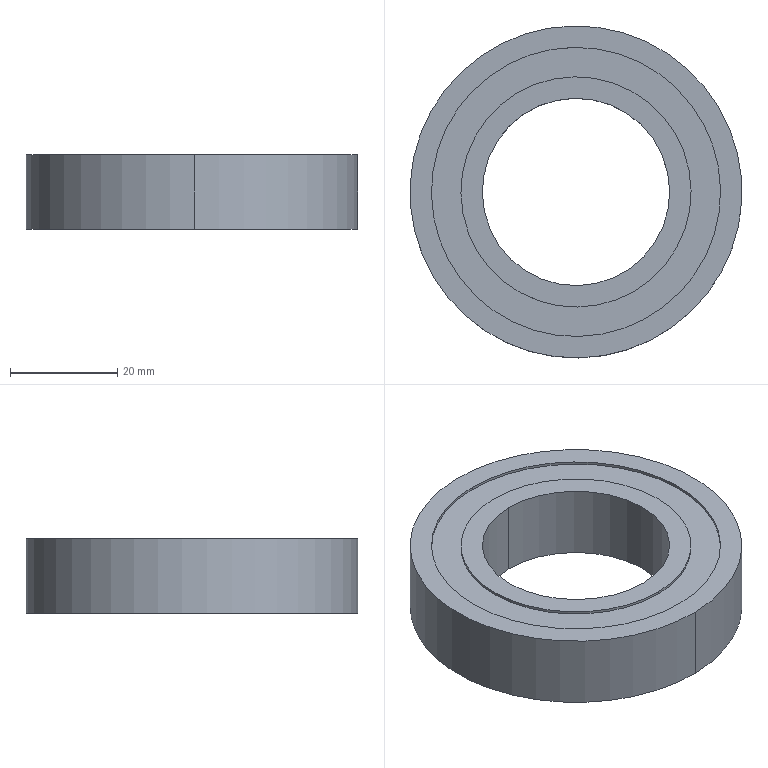Component | SolidWorks | DeepGrooveBallBearing6007-1 | 1 solid | 18 faces | box 62 x 62 x 14 mm | volume 27959 mm3 | cylinder 12 | plane 6 | commonest cylinder face diameters 54 x4 43 x4 62 x2 35 x2 | material A3
build123d program:
from build123d import *


with BuildPart() as part:
    # Sketch1 → Revolve1 (revolve)
    with BuildSketch(Plane(origin=(0, 0, 0), x_dir=(1, 0, 0), z_dir=(0, 1, 0)), mode=Mode.PRIVATE) as revolve1_sk:
        Polygon((-31, -7), (-31, 7), (-27, 7), (-27, 6.5), (-21.5, 6.5), (-21.5, 7), (-17.5, 7), (-17.5, -7), (-21.5, -7), (-21.5, -6.5), (-27, -6.5), (-27, -7), align=None)
    revolve(revolve1_sk.sketch.rotate(Axis((0, 0, 0), (0, 0, -1)), 180), axis=Axis((0, 0, 0), (0, 0, -1)))


solid = part.part

# Placed as in the assembly
solid = solid.moved(Location((733.029, 200.722, 14.5), (0, 0, 0)))
STEP:
#1=COLOUR_RGB('',0.7922,0.8196,0.9333);
#2=FILL_AREA_STYLE_COLOUR('',#1);
#3=FILL_AREA_STYLE('',(#2));
#4=SURFACE_STYLE_FILL_AREA(#3);
#5=SURFACE_SIDE_STYLE('',(#4));
#6=SURFACE_STYLE_USAGE(.BOTH.,#5);
#7=PRESENTATION_STYLE_ASSIGNMENT((#6));
#8=CARTESIAN_POINT('',(28.879,6.682,0.8465));
#9=VERTEX_POINT('',#8);
#10=CARTESIAN_POINT('',(28.839,9.123,0.8465));
#11=VERTEX_POINT('',#10);
#12=CARTESIAN_POINT('',(28.859,7.902,0.8465));
#13=DIRECTION('',(-0.,-0.,-1.));
#14=DIRECTION('',(0.01645,-0.9999,0.));
#15=AXIS2_PLACEMENT_3D('',#12,#13,#14);
#16=CIRCLE('',#15,1.22);
#17=EDGE_CURVE('',#9,#11,#16,.T.);
#18=ORIENTED_EDGE('',*,*,#17,.T.);
#19=CARTESIAN_POINT('',(28.839,9.123,0.2953));
#20=VERTEX_POINT('',#19);
#21=CARTESIAN_POINT('',(28.839,9.123,0.5709));
#22=DIRECTION('',(-0.,-0.,-1.));
#23=VECTOR('',#22,39.37);
#24=LINE('',#21,#23);
#25=EDGE_CURVE('',#11,#20,#24,.T.);
#26=ORIENTED_EDGE('',*,*,#25,.T.);
#27=CARTESIAN_POINT('',(28.879,6.682,0.2953));
#28=VERTEX_POINT('',#27);
#29=CARTESIAN_POINT('',(28.859,7.902,0.2953));
#30=DIRECTION('',(-0.,-0.,-1.));
#31=DIRECTION('',(0.01645,-0.9999,0.));
#32=AXIS2_PLACEMENT_3D('',#29,#30,#31);
#33=CIRCLE('',#32,1.22);
#34=EDGE_CURVE('',#28,#20,#33,.T.);
#35=ORIENTED_EDGE('',*,*,#34,.F.);
#36=CARTESIAN_POINT('',(28.879,6.682,0.5709));
#37=DIRECTION('',(-0.,-0.,-1.));
#38=VECTOR('',#37,39.37);
#39=LINE('',#36,#38);
#40=EDGE_CURVE('',#9,#28,#39,.T.);
#41=ORIENTED_EDGE('',*,*,#40,.F.);
#42=EDGE_LOOP('',(#18,#26,#35,#41));
#43=FACE_OUTER_BOUND('',#42,.T.);
#44=CARTESIAN_POINT('',(28.859,7.902,0.5709));
#45=DIRECTION('',(-0.,-0.,-1.));
#46=DIRECTION('',(0.01645,-0.9999,0.));
#47=AXIS2_PLACEMENT_3D('',#44,#45,#46);
#48=CYLINDRICAL_SURFACE('',#47,1.22);
#49=ADVANCED_FACE('',(#43),#48,.T.);
#50=CARTESIAN_POINT('',(28.842,8.965,0.315));
#51=VERTEX_POINT('',#50);
#52=CARTESIAN_POINT('',(28.877,6.84,0.315));
#53=VERTEX_POINT('',#52);
#54=CARTESIAN_POINT('',(28.859,7.902,0.315));
#55=DIRECTION('',(-0.,-0.,-1.));
#56=DIRECTION('',(0.01645,-0.9999,0.));
#57=AXIS2_PLACEMENT_3D('',#54,#55,#56);
#58=CIRCLE('',#57,1.063);
#59=EDGE_CURVE('',#51,#53,#58,.T.);
#60=ORIENTED_EDGE('',*,*,#59,.F.);
#61=CARTESIAN_POINT('',(28.842,8.965,0.2953));
#62=VERTEX_POINT('',#61);
#63=CARTESIAN_POINT('',(28.842,8.965,0.5709));
#64=DIRECTION('',(-0.,-0.,-1.));
#65=VECTOR('',#64,39.37);
#66=LINE('',#63,#65);
#67=EDGE_CURVE('',#51,#62,#66,.T.);
#68=ORIENTED_EDGE('',*,*,#67,.T.);
#69=CARTESIAN_POINT('',(28.877,6.84,0.2953));
#70=VERTEX_POINT('',#69);
#71=CARTESIAN_POINT('',(28.859,7.902,0.2953));
#72=DIRECTION('',(-0.,-0.,-1.));
#73=DIRECTION('',(0.01645,-0.9999,0.));
#74=AXIS2_PLACEMENT_3D('',#71,#72,#73);
#75=CIRCLE('',#74,1.063);
#76=EDGE_CURVE('',#62,#70,#75,.T.);
#77=ORIENTED_EDGE('',*,*,#76,.T.);
#78=CARTESIAN_POINT('',(28.877,6.84,0.5709));
#79=DIRECTION('',(-0.,-0.,-1.));
#80=VECTOR('',#79,39.37);
#81=LINE('',#78,#80);
#82=EDGE_CURVE('',#53,#70,#81,.T.);
#83=ORIENTED_EDGE('',*,*,#82,.F.);
#84=EDGE_LOOP('',(#60,#68,#77,#83));
#85=FACE_OUTER_BOUND('',#84,.T.);
#86=CARTESIAN_POINT('',(28.859,7.902,0.5709));
#87=DIRECTION('',(-0.,-0.,-1.));
#88=DIRECTION('',(0.01645,-0.9999,0.));
#89=AXIS2_PLACEMENT_3D('',#86,#87,#88);
#90=CYLINDRICAL_SURFACE('',#89,1.063);
#91=ADVANCED_FACE('',(#85),#90,.F.);
#92=CARTESIAN_POINT('',(28.873,7.056,0.315));
#93=VERTEX_POINT('',#92);
#94=CARTESIAN_POINT('',(28.845,8.749,0.315));
#95=VERTEX_POINT('',#94);
#96=CARTESIAN_POINT('',(28.859,7.902,0.315));
#97=DIRECTION('',(-0.,-0.,-1.));
#98=DIRECTION('',(0.01645,-0.9999,0.));
#99=AXIS2_PLACEMENT_3D('',#96,#97,#98);
#100=CIRCLE('',#99,0.8465);
#101=EDGE_CURVE('',#93,#95,#100,.T.);
#102=ORIENTED_EDGE('',*,*,#101,.T.);
#103=CARTESIAN_POINT('',(28.845,8.749,0.2953));
#104=VERTEX_POINT('',#103);
#105=CARTESIAN_POINT('',(28.845,8.749,0.5709));
#106=DIRECTION('',(-0.,-0.,-1.));
#107=VECTOR('',#106,39.37);
#108=LINE('',#105,#107);
#109=EDGE_CURVE('',#95,#104,#108,.T.);
#110=ORIENTED_EDGE('',*,*,#109,.T.);
#111=CARTESIAN_POINT('',(28.873,7.056,0.2953));
#112=VERTEX_POINT('',#111);
#113=CARTESIAN_POINT('',(28.859,7.902,0.2953));
#114=DIRECTION('',(-0.,-0.,-1.));
#115=DIRECTION('',(0.01645,-0.9999,0.));
#116=AXIS2_PLACEMENT_3D('',#113,#114,#115);
#117=CIRCLE('',#116,0.8465);
#118=EDGE_CURVE('',#112,#104,#117,.T.);
#119=ORIENTED_EDGE('',*,*,#118,.F.);
#120=CARTESIAN_POINT('',(28.873,7.056,0.5709));
#121=DIRECTION('',(-0.,-0.,-1.));
#122=VECTOR('',#121,39.37);
#123=LINE('',#120,#122);
#124=EDGE_CURVE('',#93,#112,#123,.T.);
#125=ORIENTED_EDGE('',*,*,#124,.F.);
#126=EDGE_LOOP('',(#102,#110,#119,#125));
#127=FACE_OUTER_BOUND('',#126,.T.);
#128=CARTESIAN_POINT('',(28.859,7.902,0.5709));
#129=DIRECTION('',(-0.,-0.,-1.));
#130=DIRECTION('',(0.01645,-0.9999,0.));
#131=AXIS2_PLACEMENT_3D('',#128,#129,#130);
#132=CYLINDRICAL_SURFACE('',#131,0.8465);
#133=ADVANCED_FACE('',(#127),#132,.T.);
#134=CARTESIAN_POINT('',(28.848,8.591,0.8465));
#135=VERTEX_POINT('',#134);
#136=CARTESIAN_POINT('',(28.871,7.214,0.8465));
#137=VERTEX_POINT('',#136);
#138=CARTESIAN_POINT('',(28.859,7.902,0.8465));
#139=DIRECTION('',(-0.,-0.,-1.));
#140=DIRECTION('',(0.01645,-0.9999,0.));
#141=AXIS2_PLACEMENT_3D('',#138,#139,#140);
#142=CIRCLE('',#141,0.689);
#143=EDGE_CURVE('',#135,#137,#142,.T.);
#144=ORIENTED_EDGE('',*,*,#143,.F.);
#145=CARTESIAN_POINT('',(28.848,8.591,0.2953));
#146=VERTEX_POINT('',#145);
#147=CARTESIAN_POINT('',(28.848,8.591,0.5709));
#148=DIRECTION('',(-0.,-0.,-1.));
#149=VECTOR('',#148,39.37);
#150=LINE('',#147,#149);
#151=EDGE_CURVE('',#135,#146,#150,.T.);
#152=ORIENTED_EDGE('',*,*,#151,.T.);
#153=CARTESIAN_POINT('',(28.871,7.214,0.2953));
#154=VERTEX_POINT('',#153);
#155=CARTESIAN_POINT('',(28.859,7.902,0.2953));
#156=DIRECTION('',(-0.,-0.,-1.));
#157=DIRECTION('',(0.01645,-0.9999,0.));
#158=AXIS2_PLACEMENT_3D('',#155,#156,#157);
#159=CIRCLE('',#158,0.689);
#160=EDGE_CURVE('',#146,#154,#159,.T.);
#161=ORIENTED_EDGE('',*,*,#160,.T.);
#162=CARTESIAN_POINT('',(28.871,7.214,0.5709));
#163=DIRECTION('',(-0.,-0.,-1.));
#164=VECTOR('',#163,39.37);
#165=LINE('',#162,#164);
#166=EDGE_CURVE('',#137,#154,#165,.T.);
#167=ORIENTED_EDGE('',*,*,#166,.F.);
#168=EDGE_LOOP('',(#144,#152,#161,#167));
#169=FACE_OUTER_BOUND('',#168,.T.);
#170=CARTESIAN_POINT('',(28.859,7.902,0.5709));
#171=DIRECTION('',(-0.,-0.,-1.));
#172=DIRECTION('',(0.01645,-0.9999,0.));
#173=AXIS2_PLACEMENT_3D('',#170,#171,#172);
#174=CYLINDRICAL_SURFACE('',#173,0.689);
#175=ADVANCED_FACE('',(#169),#174,.F.);
#176=CARTESIAN_POINT('',(28.873,7.056,0.8465));
#177=VERTEX_POINT('',#176);
#178=CARTESIAN_POINT('',(28.845,8.749,0.8465));
#179=VERTEX_POINT('',#178);
#180=CARTESIAN_POINT('',(28.859,7.902,0.8465));
#181=DIRECTION('',(-0.,-0.,-1.));
#182=DIRECTION('',(0.01645,-0.9999,0.));
#183=AXIS2_PLACEMENT_3D('',#180,#181,#182);
#184=CIRCLE('',#183,0.8465);
#185=EDGE_CURVE('',#177,#179,#184,.T.);
#186=ORIENTED_EDGE('',*,*,#185,.T.);
#187=CARTESIAN_POINT('',(28.845,8.749,0.8268));
#188=VERTEX_POINT('',#187);
#189=CARTESIAN_POINT('',(28.845,8.749,0.5709));
#190=DIRECTION('',(-0.,-0.,-1.));
#191=VECTOR('',#190,39.37);
#192=LINE('',#189,#191);
#193=EDGE_CURVE('',#179,#188,#192,.T.);
#194=ORIENTED_EDGE('',*,*,#193,.T.);
#195=CARTESIAN_POINT('',(28.873,7.056,0.8268));
#196=VERTEX_POINT('',#195);
#197=CARTESIAN_POINT('',(28.859,7.902,0.8268));
#198=DIRECTION('',(-0.,-0.,-1.));
#199=DIRECTION('',(0.01645,-0.9999,0.));
#200=AXIS2_PLACEMENT_3D('',#197,#198,#199);
#201=CIRCLE('',#200,0.8465);
#202=EDGE_CURVE('',#196,#188,#201,.T.);
#203=ORIENTED_EDGE('',*,*,#202,.F.);
#204=CARTESIAN_POINT('',(28.873,7.056,0.5709));
#205=DIRECTION('',(-0.,-0.,-1.));
#206=VECTOR('',#205,39.37);
#207=LINE('',#204,#206);
#208=EDGE_CURVE('',#177,#196,#207,.T.);
#209=ORIENTED_EDGE('',*,*,#208,.F.);
#210=EDGE_LOOP('',(#186,#194,#203,#209));
#211=FACE_OUTER_BOUND('',#210,.T.);
#212=CARTESIAN_POINT('',(28.859,7.902,0.5709));
#213=DIRECTION('',(-0.,-0.,-1.));
#214=DIRECTION('',(0.01645,-0.9999,0.));
#215=AXIS2_PLACEMENT_3D('',#212,#213,#214);
#216=CYLINDRICAL_SURFACE('',#215,0.8465);
#217=ADVANCED_FACE('',(#211),#216,.T.);
#218=CARTESIAN_POINT('',(28.842,8.965,0.8465));
#219=VERTEX_POINT('',#218);
#220=CARTESIAN_POINT('',(28.877,6.84,0.8465));
#221=VERTEX_POINT('',#220);
#222=CARTESIAN_POINT('',(28.859,7.902,0.8465));
#223=DIRECTION('',(-0.,-0.,-1.));
#224=DIRECTION('',(0.01645,-0.9999,0.));
#225=AXIS2_PLACEMENT_3D('',#222,#223,#224);
#226=CIRCLE('',#225,1.063);
#227=EDGE_CURVE('',#219,#221,#226,.T.);
#228=ORIENTED_EDGE('',*,*,#227,.F.);
#229=CARTESIAN_POINT('',(28.842,8.965,0.8268));
#230=VERTEX_POINT('',#229);
#231=CARTESIAN_POINT('',(28.842,8.965,0.5709));
#232=DIRECTION('',(-0.,-0.,-1.));
#233=VECTOR('',#232,39.37);
#234=LINE('',#231,#233);
#235=EDGE_CURVE('',#219,#230,#234,.T.);
#236=ORIENTED_EDGE('',*,*,#235,.T.);
#237=CARTESIAN_POINT('',(28.877,6.84,0.8268));
#238=VERTEX_POINT('',#237);
#239=CARTESIAN_POINT('',(28.859,7.902,0.8268));
#240=DIRECTION('',(-0.,-0.,-1.));
#241=DIRECTION('',(0.01645,-0.9999,0.));
#242=AXIS2_PLACEMENT_3D('',#239,#240,#241);
#243=CIRCLE('',#242,1.063);
#244=EDGE_CURVE('',#230,#238,#243,.T.);
#245=ORIENTED_EDGE('',*,*,#244,.T.);
#246=CARTESIAN_POINT('',(28.877,6.84,0.5709));
#247=DIRECTION('',(-0.,-0.,-1.));
#248=VECTOR('',#247,39.37);
#249=LINE('',#246,#248);
#250=EDGE_CURVE('',#221,#238,#249,.T.);
#251=ORIENTED_EDGE('',*,*,#250,.F.);
#252=EDGE_LOOP('',(#228,#236,#245,#251));
#253=FACE_OUTER_BOUND('',#252,.T.);
#254=CARTESIAN_POINT('',(28.859,7.902,0.5709));
#255=DIRECTION('',(-0.,-0.,-1.));
#256=DIRECTION('',(0.01645,-0.9999,0.));
#257=AXIS2_PLACEMENT_3D('',#254,#255,#256);
#258=CYLINDRICAL_SURFACE('',#257,1.063);
#259=ADVANCED_FACE('',(#253),#258,.F.);
#260=ORIENTED_EDGE('',*,*,#17,.F.);
#261=CARTESIAN_POINT('',(28.859,7.902,0.8465));
#262=DIRECTION('',(-0.,-0.,-1.));
#263=DIRECTION('',(0.01645,-0.9999,0.));
#264=AXIS2_PLACEMENT_3D('',#261,#262,#263);
#265=CIRCLE('',#264,1.22);
#266=EDGE_CURVE('',#11,#9,#265,.T.);
#267=ORIENTED_EDGE('',*,*,#266,.F.);
#268=EDGE_LOOP('',(#260,#267));
#269=FACE_OUTER_BOUND('',#268,.T.);
#270=CARTESIAN_POINT('',(28.859,7.902,0.8465));
#271=DIRECTION('',(-0.,-0.,-1.));
#272=DIRECTION('',(0.01645,-0.9999,0.));
#273=AXIS2_PLACEMENT_3D('',#270,#271,#272);
#274=CIRCLE('',#273,1.063);
#275=EDGE_CURVE('',#221,#219,#274,.T.);
#276=ORIENTED_EDGE('',*,*,#275,.T.);
#277=ORIENTED_EDGE('',*,*,#227,.T.);
#278=EDGE_LOOP('',(#276,#277));
#279=FACE_BOUND('',#278,.T.);
#280=CARTESIAN_POINT('',(28.839,9.123,0.8465));
#281=DIRECTION('',(-0.,0.,-1.));
#282=DIRECTION('',(0.01645,-0.9999,-0.));
#283=AXIS2_PLACEMENT_3D('',#280,#281,#282);
#284=PLANE('',#283);
#285=ADVANCED_FACE('',(#269,#279),#284,.F.);
#286=ORIENTED_EDGE('',*,*,#235,.F.);
#287=ORIENTED_EDGE('',*,*,#275,.F.);
#288=ORIENTED_EDGE('',*,*,#250,.T.);
#289=CARTESIAN_POINT('',(28.859,7.902,0.8268));
#290=DIRECTION('',(-0.,-0.,-1.));
#291=DIRECTION('',(0.01645,-0.9999,0.));
#292=AXIS2_PLACEMENT_3D('',#289,#290,#291);
#293=CIRCLE('',#292,1.063);
#294=EDGE_CURVE('',#238,#230,#293,.T.);
#295=ORIENTED_EDGE('',*,*,#294,.T.);
#296=EDGE_LOOP('',(#286,#287,#288,#295));
#297=FACE_OUTER_BOUND('',#296,.T.);
#298=CARTESIAN_POINT('',(28.859,7.902,0.5709));
#299=DIRECTION('',(-0.,-0.,-1.));
#300=DIRECTION('',(0.01645,-0.9999,0.));
#301=AXIS2_PLACEMENT_3D('',#298,#299,#300);
#302=CYLINDRICAL_SURFACE('',#301,1.063);
#303=ADVANCED_FACE('',(#297),#302,.F.);
#304=ORIENTED_EDGE('',*,*,#294,.F.);
#305=ORIENTED_EDGE('',*,*,#244,.F.);
#306=EDGE_LOOP('',(#304,#305));
#307=FACE_OUTER_BOUND('',#306,.T.);
#308=ORIENTED_EDGE('',*,*,#202,.T.);
#309=CARTESIAN_POINT('',(28.859,7.902,0.8268));
#310=DIRECTION('',(-0.,-0.,-1.));
#311=DIRECTION('',(0.01645,-0.9999,0.));
#312=AXIS2_PLACEMENT_3D('',#309,#310,#311);
#313=CIRCLE('',#312,0.8465);
#314=EDGE_CURVE('',#188,#196,#313,.T.);
#315=ORIENTED_EDGE('',*,*,#314,.T.);
#316=EDGE_LOOP('',(#308,#315));
#317=FACE_BOUND('',#316,.T.);
#318=CARTESIAN_POINT('',(28.842,8.965,0.8268));
#319=DIRECTION('',(-0.,0.,-1.));
#320=DIRECTION('',(0.01645,-0.9999,-0.));
#321=AXIS2_PLACEMENT_3D('',#318,#319,#320);
#322=PLANE('',#321);
#323=ADVANCED_FACE('',(#307,#317),#322,.F.);
#324=ORIENTED_EDGE('',*,*,#193,.F.);
#325=CARTESIAN_POINT('',(28.859,7.902,0.8465));
#326=DIRECTION('',(-0.,-0.,-1.));
#327=DIRECTION('',(0.01645,-0.9999,0.));
#328=AXIS2_PLACEMENT_3D('',#325,#326,#327);
#329=CIRCLE('',#328,0.8465);
#330=EDGE_CURVE('',#179,#177,#329,.T.);
#331=ORIENTED_EDGE('',*,*,#330,.T.);
#332=ORIENTED_EDGE('',*,*,#208,.T.);
#333=ORIENTED_EDGE('',*,*,#314,.F.);
#334=EDGE_LOOP('',(#324,#331,#332,#333));
#335=FACE_OUTER_BOUND('',#334,.T.);
#336=CARTESIAN_POINT('',(28.859,7.902,0.5709));
#337=DIRECTION('',(-0.,-0.,-1.));
#338=DIRECTION('',(0.01645,-0.9999,0.));
#339=AXIS2_PLACEMENT_3D('',#336,#337,#338);
#340=CYLINDRICAL_SURFACE('',#339,0.8465);
#341=ADVANCED_FACE('',(#335),#340,.T.);
#342=ORIENTED_EDGE('',*,*,#185,.F.);
#343=ORIENTED_EDGE('',*,*,#330,.F.);
#344=EDGE_LOOP('',(#342,#343));
#345=FACE_OUTER_BOUND('',#344,.T.);
#346=CARTESIAN_POINT('',(28.859,7.902,0.8465));
#347=DIRECTION('',(-0.,-0.,-1.));
#348=DIRECTION('',(0.01645,-0.9999,0.));
#349=AXIS2_PLACEMENT_3D('',#346,#347,#348);
#350=CIRCLE('',#349,0.689);
#351=EDGE_CURVE('',#137,#135,#350,.T.);
#352=ORIENTED_EDGE('',*,*,#351,.T.);
#353=ORIENTED_EDGE('',*,*,#143,.T.);
#354=EDGE_LOOP('',(#352,#353));
#355=FACE_BOUND('',#354,.T.);
#356=CARTESIAN_POINT('',(28.845,8.749,0.8465));
#357=DIRECTION('',(-0.,0.,-1.));
#358=DIRECTION('',(0.01645,-0.9999,-0.));
#359=AXIS2_PLACEMENT_3D('',#356,#357,#358);
#360=PLANE('',#359);
#361=ADVANCED_FACE('',(#345,#355),#360,.F.);
#362=ORIENTED_EDGE('',*,*,#151,.F.);
#363=ORIENTED_EDGE('',*,*,#351,.F.);
#364=ORIENTED_EDGE('',*,*,#166,.T.);
#365=CARTESIAN_POINT('',(28.859,7.902,0.2953));
#366=DIRECTION('',(-0.,-0.,-1.));
#367=DIRECTION('',(0.01645,-0.9999,0.));
#368=AXIS2_PLACEMENT_3D('',#365,#366,#367);
#369=CIRCLE('',#368,0.689);
#370=EDGE_CURVE('',#154,#146,#369,.T.);
#371=ORIENTED_EDGE('',*,*,#370,.T.);
#372=EDGE_LOOP('',(#362,#363,#364,#371));
#373=FACE_OUTER_BOUND('',#372,.T.);
#374=CARTESIAN_POINT('',(28.859,7.902,0.5709));
#375=DIRECTION('',(-0.,-0.,-1.));
#376=DIRECTION('',(0.01645,-0.9999,0.));
#377=AXIS2_PLACEMENT_3D('',#374,#375,#376);
#378=CYLINDRICAL_SURFACE('',#377,0.689);
#379=ADVANCED_FACE('',(#373),#378,.F.);
#380=ORIENTED_EDGE('',*,*,#370,.F.);
#381=ORIENTED_EDGE('',*,*,#160,.F.);
#382=EDGE_LOOP('',(#380,#381));
#383=FACE_BOUND('',#382,.T.);
#384=ORIENTED_EDGE('',*,*,#118,.T.);
#385=CARTESIAN_POINT('',(28.859,7.902,0.2953));
#386=DIRECTION('',(-0.,-0.,-1.));
#387=DIRECTION('',(0.01645,-0.9999,0.));
#388=AXIS2_PLACEMENT_3D('',#385,#386,#387);
#389=CIRCLE('',#388,0.8465);
#390=EDGE_CURVE('',#104,#112,#389,.T.);
#391=ORIENTED_EDGE('',*,*,#390,.T.);
#392=EDGE_LOOP('',(#384,#391));
#393=FACE_OUTER_BOUND('',#392,.T.);
#394=CARTESIAN_POINT('',(28.845,8.749,0.2953));
#395=DIRECTION('',(0.,-0.,1.));
#396=DIRECTION('',(-0.01645,0.9999,0.));
#397=AXIS2_PLACEMENT_3D('',#394,#395,#396);
#398=PLANE('',#397);
#399=ADVANCED_FACE('',(#383,#393),#398,.F.);
#400=ORIENTED_EDGE('',*,*,#109,.F.);
#401=CARTESIAN_POINT('',(28.859,7.902,0.315));
#402=DIRECTION('',(-0.,-0.,-1.));
#403=DIRECTION('',(0.01645,-0.9999,0.));
#404=AXIS2_PLACEMENT_3D('',#401,#402,#403);
#405=CIRCLE('',#404,0.8465);
#406=EDGE_CURVE('',#95,#93,#405,.T.);
#407=ORIENTED_EDGE('',*,*,#406,.T.);
#408=ORIENTED_EDGE('',*,*,#124,.T.);
#409=ORIENTED_EDGE('',*,*,#390,.F.);
#410=EDGE_LOOP('',(#400,#407,#408,#409));
#411=FACE_OUTER_BOUND('',#410,.T.);
#412=CARTESIAN_POINT('',(28.859,7.902,0.5709));
#413=DIRECTION('',(-0.,-0.,-1.));
#414=DIRECTION('',(0.01645,-0.9999,0.));
#415=AXIS2_PLACEMENT_3D('',#412,#413,#414);
#416=CYLINDRICAL_SURFACE('',#415,0.8465);
#417=ADVANCED_FACE('',(#411),#416,.T.);
#418=ORIENTED_EDGE('',*,*,#101,.F.);
#419=ORIENTED_EDGE('',*,*,#406,.F.);
#420=EDGE_LOOP('',(#418,#419));
#421=FACE_BOUND('',#420,.T.);
#422=CARTESIAN_POINT('',(28.859,7.902,0.315));
#423=DIRECTION('',(-0.,-0.,-1.));
#424=DIRECTION('',(0.01645,-0.9999,0.));
#425=AXIS2_PLACEMENT_3D('',#422,#423,#424);
#426=CIRCLE('',#425,1.063);
#427=EDGE_CURVE('',#53,#51,#426,.T.);
#428=ORIENTED_EDGE('',*,*,#427,.T.);
#429=ORIENTED_EDGE('',*,*,#59,.T.);
#430=EDGE_LOOP('',(#428,#429));
#431=FACE_OUTER_BOUND('',#430,.T.);
#432=CARTESIAN_POINT('',(28.842,8.965,0.315));
#433=DIRECTION('',(0.,-0.,1.));
#434=DIRECTION('',(-0.01645,0.9999,0.));
#435=AXIS2_PLACEMENT_3D('',#432,#433,#434);
#436=PLANE('',#435);
#437=ADVANCED_FACE('',(#421,#431),#436,.F.);
#438=ORIENTED_EDGE('',*,*,#67,.F.);
#439=ORIENTED_EDGE('',*,*,#427,.F.);
#440=ORIENTED_EDGE('',*,*,#82,.T.);
#441=CARTESIAN_POINT('',(28.859,7.902,0.2953));
#442=DIRECTION('',(-0.,-0.,-1.));
#443=DIRECTION('',(0.01645,-0.9999,0.));
#444=AXIS2_PLACEMENT_3D('',#441,#442,#443);
#445=CIRCLE('',#444,1.063);
#446=EDGE_CURVE('',#70,#62,#445,.T.);
#447=ORIENTED_EDGE('',*,*,#446,.T.);
#448=EDGE_LOOP('',(#438,#439,#440,#447));
#449=FACE_OUTER_BOUND('',#448,.T.);
#450=CARTESIAN_POINT('',(28.859,7.902,0.5709));
#451=DIRECTION('',(-0.,-0.,-1.));
#452=DIRECTION('',(0.01645,-0.9999,0.));
#453=AXIS2_PLACEMENT_3D('',#450,#451,#452);
#454=CYLINDRICAL_SURFACE('',#453,1.063);
#455=ADVANCED_FACE('',(#449),#454,.F.);
#456=ORIENTED_EDGE('',*,*,#446,.F.);
#457=ORIENTED_EDGE('',*,*,#76,.F.);
#458=EDGE_LOOP('',(#456,#457));
#459=FACE_BOUND('',#458,.T.);
#460=ORIENTED_EDGE('',*,*,#34,.T.);
#461=CARTESIAN_POINT('',(28.859,7.902,0.2953));
#462=DIRECTION('',(-0.,-0.,-1.));
#463=DIRECTION('',(0.01645,-0.9999,0.));
#464=AXIS2_PLACEMENT_3D('',#461,#462,#463);
#465=CIRCLE('',#464,1.22);
#466=EDGE_CURVE('',#20,#28,#465,.T.);
#467=ORIENTED_EDGE('',*,*,#466,.T.);
#468=EDGE_LOOP('',(#460,#467));
#469=FACE_OUTER_BOUND('',#468,.T.);
#470=CARTESIAN_POINT('',(28.839,9.123,0.2953));
#471=DIRECTION('',(0.,-0.,1.));
#472=DIRECTION('',(-0.01645,0.9999,0.));
#473=AXIS2_PLACEMENT_3D('',#470,#471,#472);
#474=PLANE('',#473);
#475=ADVANCED_FACE('',(#459,#469),#474,.F.);
#476=ORIENTED_EDGE('',*,*,#25,.F.);
#477=ORIENTED_EDGE('',*,*,#266,.T.);
#478=ORIENTED_EDGE('',*,*,#40,.T.);
#479=ORIENTED_EDGE('',*,*,#466,.F.);
#480=EDGE_LOOP('',(#476,#477,#478,#479));
#481=FACE_OUTER_BOUND('',#480,.T.);
#482=CARTESIAN_POINT('',(28.859,7.902,0.5709));
#483=DIRECTION('',(-0.,-0.,-1.));
#484=DIRECTION('',(0.01645,-0.9999,0.));
#485=AXIS2_PLACEMENT_3D('',#482,#483,#484);
#486=CYLINDRICAL_SURFACE('',#485,1.22);
#487=ADVANCED_FACE('',(#481),#486,.T.);
#488=CLOSED_SHELL('',(#49,#91,#133,#175,#217,#259,#285,#303,#323,#341,#361,#379,#399,#417,#437,#455,#475,#487));
#489=MANIFOLD_SOLID_BREP('',#488);
#490=STYLED_ITEM('',(#7),#489);
#491=PRESENTATION_LAYER_ASSIGNMENT('','',(#490));
#492=(LENGTH_UNIT()NAMED_UNIT(*)SI_UNIT($,.METRE.));
#493=LENGTH_MEASURE_WITH_UNIT(LENGTH_MEASURE(0.0254),#492);
#494=DIMENSIONAL_EXPONENTS(1.,0.,0.,0.,0.,0.,0.);
#495=(CONVERSION_BASED_UNIT('',#493)LENGTH_UNIT()NAMED_UNIT(#494));
#496=UNCERTAINTY_MEASURE_WITH_UNIT(LENGTH_MEASURE(0.00001),#495,'','');
#497=(NAMED_UNIT(*)PLANE_ANGLE_UNIT()SI_UNIT($,.RADIAN.));
#498=(NAMED_UNIT(*)SI_UNIT($,.STERADIAN.)SOLID_ANGLE_UNIT());
#499=(GEOMETRIC_REPRESENTATION_CONTEXT(3)GLOBAL_UNCERTAINTY_ASSIGNED_CONTEXT((#496))GLOBAL_UNIT_ASSIGNED_CONTEXT((#495,#497,#498))REPRESENTATION_CONTEXT('',''));
#500=MECHANICAL_DESIGN_GEOMETRIC_PRESENTATION_REPRESENTATION('',(#490),#499);
#501=CARTESIAN_POINT('',(0.,0.,0.));
#502=DIRECTION('',(0.,0.,1.));
#503=DIRECTION('',(1.,0.,0.));
#504=AXIS2_PLACEMENT_3D('',#501,#502,#503);
#505=(LENGTH_UNIT()NAMED_UNIT(*)SI_UNIT($,.METRE.));
#506=LENGTH_MEASURE_WITH_UNIT(LENGTH_MEASURE(0.0254),#505);
#507=DIMENSIONAL_EXPONENTS(1.,0.,0.,0.,0.,0.,0.);
#508=(CONVERSION_BASED_UNIT('',#506)LENGTH_UNIT()NAMED_UNIT(#507));
#509=UNCERTAINTY_MEASURE_WITH_UNIT(LENGTH_MEASURE(0.00001),#508,'','');
#510=(NAMED_UNIT(*)PLANE_ANGLE_UNIT()SI_UNIT($,.RADIAN.));
#511=(NAMED_UNIT(*)SI_UNIT($,.STERADIAN.)SOLID_ANGLE_UNIT());
#512=(GEOMETRIC_REPRESENTATION_CONTEXT(3)GLOBAL_UNCERTAINTY_ASSIGNED_CONTEXT((#509))GLOBAL_UNIT_ASSIGNED_CONTEXT((#508,#510,#511))REPRESENTATION_CONTEXT('',''));
#513=ADVANCED_BREP_SHAPE_REPRESENTATION('',(#489,#504),#512);